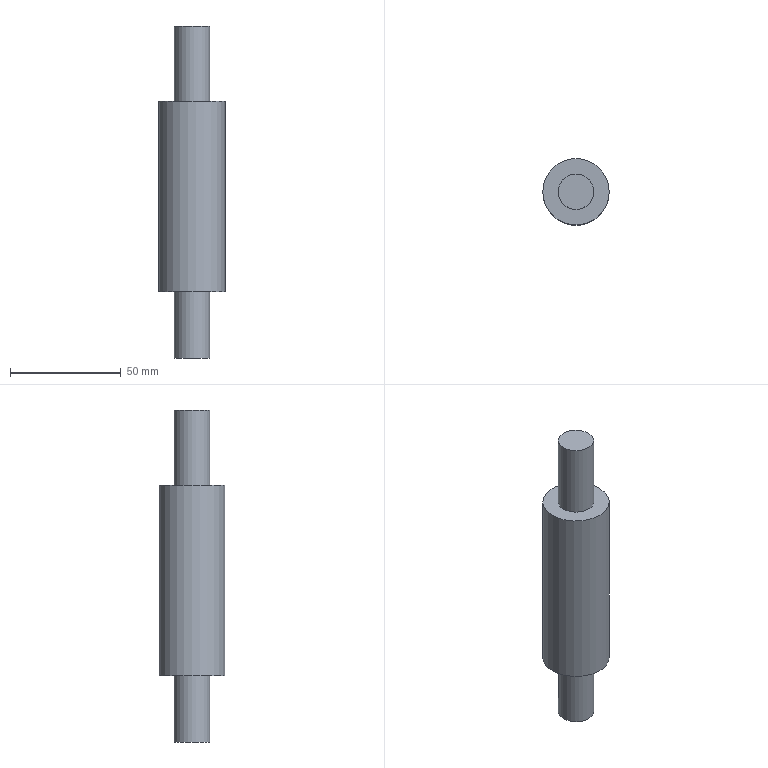Component | NX | SUPPORT_ROD | 1 solid | 7 faces | box 30 x 30 x 150 mm | volume 73658 mm3 | plane 4 | cylinder 3 | commonest cylinder face diameters 16 x2 30 x1
STEP:
#1=CARTESIAN_POINT('',(0.,0.,0.));
#2=DIRECTION('',(0.,0.,1.));
#3=DIRECTION('',(1.,0.,0.));
#4=AXIS2_PLACEMENT_3D('',#1,#2,#3);
#5=CARTESIAN_POINT('',(-85.,0.,158.));
#6=VERTEX_POINT('',#5);
#7=CARTESIAN_POINT('',(-100.,0.,158.));
#8=DIRECTION('',(0.,0.,1.));
#9=DIRECTION('',(1.,0.,0.));
#10=AXIS2_PLACEMENT_3D('',#7,#8,#9);
#11=CIRCLE('',#10,15.);
#12=CARTESIAN_POINT('',(-100.,0.,158.));
#13=DIRECTION('',(0.,0.,-1.));
#14=DIRECTION('',(-1.,0.,0.));
#15=AXIS2_PLACEMENT_3D('',#12,#13,#14);
#16=CYLINDRICAL_SURFACE('',#15,15.);
#17=CARTESIAN_POINT('',(9.425,0.));
#18=DIRECTION('',(-1.,0.));
#19=VECTOR('',#18,1.);
#20=LINE('',#17,#19);
#21=(GEOMETRIC_REPRESENTATION_CONTEXT(2)PARAMETRIC_REPRESENTATION_CONTEXT()REPRESENTATION_CONTEXT('',''));
#22=DEFINITIONAL_REPRESENTATION('',(#20),#21);
#23=PCURVE('',#16,#22);
#24=CARTESIAN_POINT('',(-100.,0.,158.));
#25=DIRECTION('',(0.,0.,1.));
#26=DIRECTION('',(1.,0.,0.));
#27=AXIS2_PLACEMENT_3D('',#24,#25,#26);
#28=PLANE('',#27);
#29=CARTESIAN_POINT('',(0.,0.));
#30=DIRECTION('',(1.,0.));
#31=AXIS2_PLACEMENT_2D('',#29,#30);
#32=CIRCLE('',#31,15.);
#33=(GEOMETRIC_REPRESENTATION_CONTEXT(2)PARAMETRIC_REPRESENTATION_CONTEXT()REPRESENTATION_CONTEXT('',''));
#34=DEFINITIONAL_REPRESENTATION('',(#32),#33);
#35=PCURVE('',#28,#34);
#36=SURFACE_CURVE('',#11,(#23,#35),.PCURVE_S1.);
#37=EDGE_CURVE('',#6,#6,#36,.T.);
#38=ORIENTED_EDGE('',*,*,#37,.F.);
#39=CARTESIAN_POINT('',(-85.,0.,72.));
#40=VERTEX_POINT('',#39);
#41=CARTESIAN_POINT('',(-85.,0.,158.));
#42=CARTESIAN_POINT('',(-85.,0.,72.));
#43=B_SPLINE_CURVE_WITH_KNOTS('',1,(#41,#42),.UNSPECIFIED.,.F.,.F.,(2,2),(0.,86.),.PIECEWISE_BEZIER_KNOTS.);
#44=CARTESIAN_POINT('',(9.425,0.));
#45=DIRECTION('',(0.,1.));
#46=VECTOR('',#45,1.);
#47=LINE('',#44,#46);
#48=(GEOMETRIC_REPRESENTATION_CONTEXT(2)PARAMETRIC_REPRESENTATION_CONTEXT()REPRESENTATION_CONTEXT('',''));
#49=DEFINITIONAL_REPRESENTATION('',(#47),#48);
#50=PCURVE('',#16,#49);
#51=CARTESIAN_POINT('',(3.142,0.));
#52=DIRECTION('',(0.,1.));
#53=VECTOR('',#52,1.);
#54=LINE('',#51,#53);
#55=(GEOMETRIC_REPRESENTATION_CONTEXT(2)PARAMETRIC_REPRESENTATION_CONTEXT()REPRESENTATION_CONTEXT('',''));
#56=DEFINITIONAL_REPRESENTATION('',(#54),#55);
#57=PCURVE('',#16,#56);
#58=SEAM_CURVE('',#43,(#50,#57),.PCURVE_S1.);
#59=EDGE_CURVE('',#6,#40,#58,.T.);
#60=ORIENTED_EDGE('',*,*,#59,.T.);
#61=CARTESIAN_POINT('',(-100.,0.,72.));
#62=DIRECTION('',(0.,0.,1.));
#63=DIRECTION('',(1.,0.,0.));
#64=AXIS2_PLACEMENT_3D('',#61,#62,#63);
#65=CIRCLE('',#64,15.);
#66=CARTESIAN_POINT('',(9.425,86.));
#67=DIRECTION('',(-1.,0.));
#68=VECTOR('',#67,1.);
#69=LINE('',#66,#68);
#70=(GEOMETRIC_REPRESENTATION_CONTEXT(2)PARAMETRIC_REPRESENTATION_CONTEXT()REPRESENTATION_CONTEXT('',''));
#71=DEFINITIONAL_REPRESENTATION('',(#69),#70);
#72=PCURVE('',#16,#71);
#73=CARTESIAN_POINT('',(-100.,0.,72.));
#74=DIRECTION('',(0.,0.,1.));
#75=DIRECTION('',(1.,0.,0.));
#76=AXIS2_PLACEMENT_3D('',#73,#74,#75);
#77=PLANE('',#76);
#78=CARTESIAN_POINT('',(0.,0.));
#79=DIRECTION('',(1.,0.));
#80=AXIS2_PLACEMENT_2D('',#78,#79);
#81=CIRCLE('',#80,15.);
#82=(GEOMETRIC_REPRESENTATION_CONTEXT(2)PARAMETRIC_REPRESENTATION_CONTEXT()REPRESENTATION_CONTEXT('',''));
#83=DEFINITIONAL_REPRESENTATION('',(#81),#82);
#84=PCURVE('',#77,#83);
#85=SURFACE_CURVE('',#65,(#72,#84),.PCURVE_S1.);
#86=EDGE_CURVE('',#40,#40,#85,.T.);
#87=ORIENTED_EDGE('',*,*,#86,.T.);
#88=ORIENTED_EDGE('',*,*,#59,.F.);
#89=EDGE_LOOP('',(#38,#60,#87,#88));
#90=FACE_BOUND('',#89,.T.);
#91=ADVANCED_FACE('',(#90),#16,.T.);
#92=CARTESIAN_POINT('',(-92.,0.,158.));
#93=VERTEX_POINT('',#92);
#94=CARTESIAN_POINT('',(-100.,0.,158.));
#95=DIRECTION('',(0.,0.,1.));
#96=DIRECTION('',(1.,0.,0.));
#97=AXIS2_PLACEMENT_3D('',#94,#95,#96);
#98=CIRCLE('',#97,8.);
#99=CARTESIAN_POINT('',(0.,0.));
#100=DIRECTION('',(1.,0.));
#101=AXIS2_PLACEMENT_2D('',#99,#100);
#102=CIRCLE('',#101,8.);
#103=(GEOMETRIC_REPRESENTATION_CONTEXT(2)PARAMETRIC_REPRESENTATION_CONTEXT()REPRESENTATION_CONTEXT('',''));
#104=DEFINITIONAL_REPRESENTATION('',(#102),#103);
#105=PCURVE('',#28,#104);
#106=CARTESIAN_POINT('',(-100.,0.,192.));
#107=DIRECTION('',(0.,0.,-1.));
#108=DIRECTION('',(-1.,0.,0.));
#109=AXIS2_PLACEMENT_3D('',#106,#107,#108);
#110=CYLINDRICAL_SURFACE('',#109,8.);
#111=CARTESIAN_POINT('',(9.425,34.));
#112=DIRECTION('',(-1.,0.));
#113=VECTOR('',#112,1.);
#114=LINE('',#111,#113);
#115=(GEOMETRIC_REPRESENTATION_CONTEXT(2)PARAMETRIC_REPRESENTATION_CONTEXT()REPRESENTATION_CONTEXT('',''));
#116=DEFINITIONAL_REPRESENTATION('',(#114),#115);
#117=PCURVE('',#110,#116);
#118=SURFACE_CURVE('',#98,(#105,#117),.PCURVE_S1.);
#119=EDGE_CURVE('',#93,#93,#118,.T.);
#120=ORIENTED_EDGE('',*,*,#119,.F.);
#121=EDGE_LOOP('',(#120));
#122=FACE_BOUND('',#121,.T.);
#123=ORIENTED_EDGE('',*,*,#37,.T.);
#124=EDGE_LOOP('',(#123));
#125=FACE_BOUND('',#124,.T.);
#126=ADVANCED_FACE('',(#122,#125),#28,.T.);
#127=CARTESIAN_POINT('',(-92.,0.,72.));
#128=VERTEX_POINT('',#127);
#129=CARTESIAN_POINT('',(-100.,0.,72.));
#130=DIRECTION('',(0.,0.,-1.));
#131=DIRECTION('',(1.,0.,0.));
#132=AXIS2_PLACEMENT_3D('',#129,#130,#131);
#133=CIRCLE('',#132,8.);
#134=CARTESIAN_POINT('',(8.,0.));
#135=CARTESIAN_POINT('',(8.,-13.856));
#136=CARTESIAN_POINT('',(-4.,-6.928));
#137=CARTESIAN_POINT('',(-16.,-0.));
#138=CARTESIAN_POINT('',(-4.,6.928));
#139=CARTESIAN_POINT('',(8.,13.856));
#140=CARTESIAN_POINT('',(8.,0.));
#141=(BOUNDED_CURVE()B_SPLINE_CURVE(2,(#134,#135,#136,#137,#138,#139,#140),.UNSPECIFIED.,.T.,.F.)B_SPLINE_CURVE_WITH_KNOTS((1,2,2,2,2,1),(-2.094,0.,2.094,4.189,6.283,8.378),.UNSPECIFIED.)CURVE()GEOMETRIC_REPRESENTATION_ITEM()RATIONAL_B_SPLINE_CURVE((1.,0.5,1.,0.5,1.,0.5,1.))REPRESENTATION_ITEM(''));
#142=(GEOMETRIC_REPRESENTATION_CONTEXT(2)PARAMETRIC_REPRESENTATION_CONTEXT()REPRESENTATION_CONTEXT('',''));
#143=DEFINITIONAL_REPRESENTATION('',(#141),#142);
#144=PCURVE('',#77,#143);
#145=CARTESIAN_POINT('',(-100.,0.,42.));
#146=DIRECTION('',(0.,0.,1.));
#147=DIRECTION('',(1.,0.,0.));
#148=AXIS2_PLACEMENT_3D('',#145,#146,#147);
#149=CYLINDRICAL_SURFACE('',#148,8.);
#150=CARTESIAN_POINT('',(6.283,30.));
#151=DIRECTION('',(-1.,0.));
#152=VECTOR('',#151,1.);
#153=LINE('',#150,#152);
#154=(GEOMETRIC_REPRESENTATION_CONTEXT(2)PARAMETRIC_REPRESENTATION_CONTEXT()REPRESENTATION_CONTEXT('',''));
#155=DEFINITIONAL_REPRESENTATION('',(#153),#154);
#156=PCURVE('',#149,#155);
#157=SURFACE_CURVE('',#133,(#144,#156),.PCURVE_S1.);
#158=EDGE_CURVE('',#128,#128,#157,.T.);
#159=ORIENTED_EDGE('',*,*,#158,.F.);
#160=EDGE_LOOP('',(#159));
#161=FACE_BOUND('',#160,.T.);
#162=ORIENTED_EDGE('',*,*,#86,.F.);
#163=EDGE_LOOP('',(#162));
#164=FACE_BOUND('',#163,.T.);
#165=ADVANCED_FACE('',(#161,#164),#77,.F.);
#166=CARTESIAN_POINT('',(-92.,0.,192.));
#167=VERTEX_POINT('',#166);
#168=CARTESIAN_POINT('',(-100.,0.,192.));
#169=DIRECTION('',(0.,0.,1.));
#170=DIRECTION('',(1.,0.,0.));
#171=AXIS2_PLACEMENT_3D('',#168,#169,#170);
#172=CIRCLE('',#171,8.);
#173=CARTESIAN_POINT('',(9.425,0.));
#174=DIRECTION('',(-1.,0.));
#175=VECTOR('',#174,1.);
#176=LINE('',#173,#175);
#177=(GEOMETRIC_REPRESENTATION_CONTEXT(2)PARAMETRIC_REPRESENTATION_CONTEXT()REPRESENTATION_CONTEXT('',''));
#178=DEFINITIONAL_REPRESENTATION('',(#176),#177);
#179=PCURVE('',#110,#178);
#180=CARTESIAN_POINT('',(-100.,0.,192.));
#181=DIRECTION('',(0.,0.,1.));
#182=DIRECTION('',(1.,0.,0.));
#183=AXIS2_PLACEMENT_3D('',#180,#181,#182);
#184=PLANE('',#183);
#185=CARTESIAN_POINT('',(0.,0.));
#186=DIRECTION('',(1.,0.));
#187=AXIS2_PLACEMENT_2D('',#185,#186);
#188=CIRCLE('',#187,8.);
#189=(GEOMETRIC_REPRESENTATION_CONTEXT(2)PARAMETRIC_REPRESENTATION_CONTEXT()REPRESENTATION_CONTEXT('',''));
#190=DEFINITIONAL_REPRESENTATION('',(#188),#189);
#191=PCURVE('',#184,#190);
#192=SURFACE_CURVE('',#172,(#179,#191),.PCURVE_S1.);
#193=EDGE_CURVE('',#167,#167,#192,.T.);
#194=ORIENTED_EDGE('',*,*,#193,.F.);
#195=CARTESIAN_POINT('',(-92.,0.,192.));
#196=CARTESIAN_POINT('',(-92.,0.,158.));
#197=B_SPLINE_CURVE_WITH_KNOTS('',1,(#195,#196),.UNSPECIFIED.,.F.,.F.,(2,2),(0.,34.),.PIECEWISE_BEZIER_KNOTS.);
#198=CARTESIAN_POINT('',(9.425,0.));
#199=DIRECTION('',(0.,1.));
#200=VECTOR('',#199,1.);
#201=LINE('',#198,#200);
#202=(GEOMETRIC_REPRESENTATION_CONTEXT(2)PARAMETRIC_REPRESENTATION_CONTEXT()REPRESENTATION_CONTEXT('',''));
#203=DEFINITIONAL_REPRESENTATION('',(#201),#202);
#204=PCURVE('',#110,#203);
#205=CARTESIAN_POINT('',(3.142,0.));
#206=DIRECTION('',(0.,1.));
#207=VECTOR('',#206,1.);
#208=LINE('',#205,#207);
#209=(GEOMETRIC_REPRESENTATION_CONTEXT(2)PARAMETRIC_REPRESENTATION_CONTEXT()REPRESENTATION_CONTEXT('',''));
#210=DEFINITIONAL_REPRESENTATION('',(#208),#209);
#211=PCURVE('',#110,#210);
#212=SEAM_CURVE('',#197,(#204,#211),.PCURVE_S1.);
#213=EDGE_CURVE('',#167,#93,#212,.T.);
#214=ORIENTED_EDGE('',*,*,#213,.T.);
#215=ORIENTED_EDGE('',*,*,#119,.T.);
#216=ORIENTED_EDGE('',*,*,#213,.F.);
#217=EDGE_LOOP('',(#194,#214,#215,#216));
#218=FACE_BOUND('',#217,.T.);
#219=ADVANCED_FACE('',(#218),#110,.T.);
#220=ORIENTED_EDGE('',*,*,#193,.T.);
#221=EDGE_LOOP('',(#220));
#222=FACE_BOUND('',#221,.T.);
#223=ADVANCED_FACE('',(#222),#184,.T.);
#224=CARTESIAN_POINT('',(-92.,0.,42.));
#225=VERTEX_POINT('',#224);
#226=CARTESIAN_POINT('',(-100.,0.,42.));
#227=DIRECTION('',(0.,0.,-1.));
#228=DIRECTION('',(1.,0.,0.));
#229=AXIS2_PLACEMENT_3D('',#226,#227,#228);
#230=CIRCLE('',#229,8.);
#231=CARTESIAN_POINT('',(6.283,0.));
#232=DIRECTION('',(-1.,0.));
#233=VECTOR('',#232,1.);
#234=LINE('',#231,#233);
#235=(GEOMETRIC_REPRESENTATION_CONTEXT(2)PARAMETRIC_REPRESENTATION_CONTEXT()REPRESENTATION_CONTEXT('',''));
#236=DEFINITIONAL_REPRESENTATION('',(#234),#235);
#237=PCURVE('',#149,#236);
#238=CARTESIAN_POINT('',(-100.,0.,42.));
#239=DIRECTION('',(0.,0.,-1.));
#240=DIRECTION('',(-1.,0.,0.));
#241=AXIS2_PLACEMENT_3D('',#238,#239,#240);
#242=PLANE('',#241);
#243=CARTESIAN_POINT('',(0.,0.));
#244=DIRECTION('',(-1.,0.));
#245=AXIS2_PLACEMENT_2D('',#243,#244);
#246=CIRCLE('',#245,8.);
#247=(GEOMETRIC_REPRESENTATION_CONTEXT(2)PARAMETRIC_REPRESENTATION_CONTEXT()REPRESENTATION_CONTEXT('',''));
#248=DEFINITIONAL_REPRESENTATION('',(#246),#247);
#249=PCURVE('',#242,#248);
#250=SURFACE_CURVE('',#230,(#237,#249),.PCURVE_S1.);
#251=EDGE_CURVE('',#225,#225,#250,.T.);
#252=ORIENTED_EDGE('',*,*,#251,.F.);
#253=CARTESIAN_POINT('',(-92.,0.,42.));
#254=CARTESIAN_POINT('',(-92.,0.,72.));
#255=B_SPLINE_CURVE_WITH_KNOTS('',1,(#253,#254),.UNSPECIFIED.,.F.,.F.,(2,2),(0.,30.),.PIECEWISE_BEZIER_KNOTS.);
#256=CARTESIAN_POINT('',(6.283,0.));
#257=DIRECTION('',(0.,1.));
#258=VECTOR('',#257,1.);
#259=LINE('',#256,#258);
#260=(GEOMETRIC_REPRESENTATION_CONTEXT(2)PARAMETRIC_REPRESENTATION_CONTEXT()REPRESENTATION_CONTEXT('',''));
#261=DEFINITIONAL_REPRESENTATION('',(#259),#260);
#262=PCURVE('',#149,#261);
#263=CARTESIAN_POINT('',(0.,0.));
#264=DIRECTION('',(0.,1.));
#265=VECTOR('',#264,1.);
#266=LINE('',#263,#265);
#267=(GEOMETRIC_REPRESENTATION_CONTEXT(2)PARAMETRIC_REPRESENTATION_CONTEXT()REPRESENTATION_CONTEXT('',''));
#268=DEFINITIONAL_REPRESENTATION('',(#266),#267);
#269=PCURVE('',#149,#268);
#270=SEAM_CURVE('',#255,(#262,#269),.PCURVE_S1.);
#271=EDGE_CURVE('',#225,#128,#270,.T.);
#272=ORIENTED_EDGE('',*,*,#271,.T.);
#273=ORIENTED_EDGE('',*,*,#158,.T.);
#274=ORIENTED_EDGE('',*,*,#271,.F.);
#275=EDGE_LOOP('',(#252,#272,#273,#274));
#276=FACE_BOUND('',#275,.T.);
#277=ADVANCED_FACE('',(#276),#149,.T.);
#278=ORIENTED_EDGE('',*,*,#251,.T.);
#279=EDGE_LOOP('',(#278));
#280=FACE_BOUND('',#279,.T.);
#281=ADVANCED_FACE('',(#280),#242,.T.);
#282=CLOSED_SHELL('',(#91,#126,#165,#219,#223,#277,#281));
#283=MANIFOLD_SOLID_BREP('',#282);
#284=(LENGTH_UNIT()NAMED_UNIT(*)SI_UNIT(.MILLI.,.METRE.));
#285=UNCERTAINTY_MEASURE_WITH_UNIT(LENGTH_MEASURE(0.00001),#284,'','');
#286=(NAMED_UNIT(*)PLANE_ANGLE_UNIT()SI_UNIT($,.RADIAN.));
#287=(NAMED_UNIT(*)SI_UNIT($,.STERADIAN.)SOLID_ANGLE_UNIT());
#288=(GEOMETRIC_REPRESENTATION_CONTEXT(3)GLOBAL_UNCERTAINTY_ASSIGNED_CONTEXT((#285))GLOBAL_UNIT_ASSIGNED_CONTEXT((#284,#286,#287))REPRESENTATION_CONTEXT('',''));
#289=ADVANCED_BREP_SHAPE_REPRESENTATION('',(#4,#283),#288);